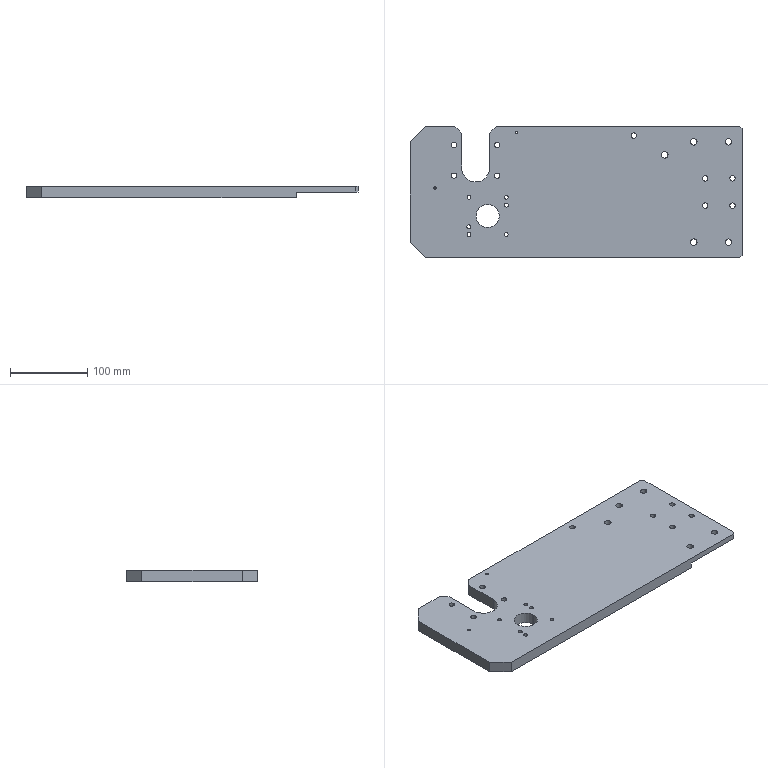Component | SolidWorks | BottomPlate(2)-1 | 1 solid | 91 faces | volume 929537 mm3 | cylinder 57 | plane 22 | cone 12 | commonest cylinder face diameters 7 x18 5 x12 11 x10 8.5 x10 3 x4 30 x2 36 x1